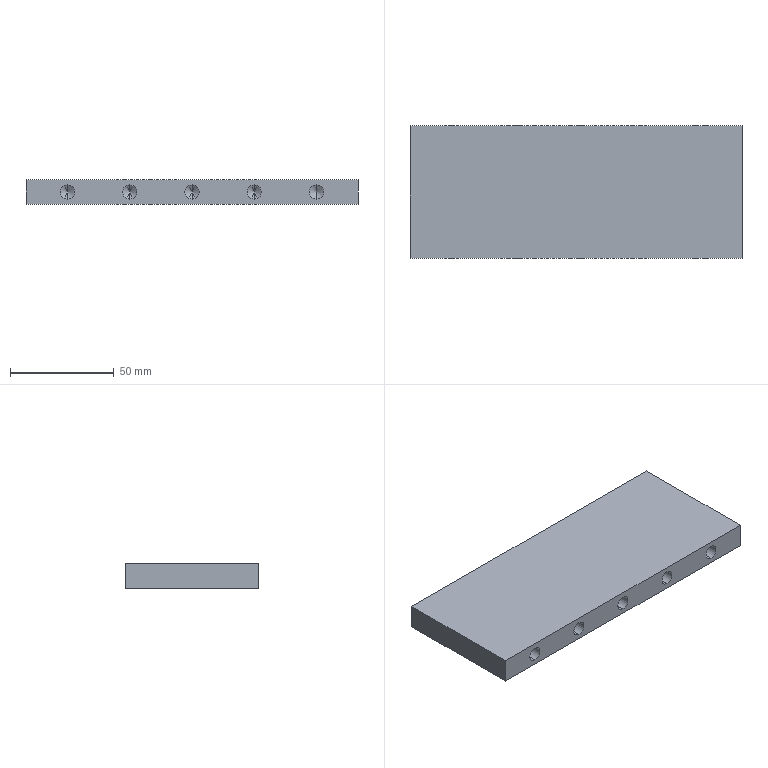Component | SolidWorks | SupportPlate2-3 | 1 solid | 46 faces | box 160 x 64 x 12 mm | volume 114552 mm3 | cylinder 20 | cone 20 | plane 6 | commonest cylinder face diameters 6.8 x20
build123d program:
from build123d import *

# Parameters (mm, degrees)
SKETCH1_W                  = 160
SKETCH1_H                  = 64
EXTRUDE1_DEPTH             = 6
M8_TAPPED_HOLE1_AT_2_COUNT = 2
M8_TAPPED_HOLE1_AT_2_PITCH = 60
M8_TAPPED_HOLE1_AT_3_COUNT = 2
M8_TAPPED_HOLE1_AT_3_PITCH = 90
M8_TAPPED_HOLE1_AT_4_COUNT = 2
M8_TAPPED_HOLE1_AT_4_PITCH = 30
M8_TAPPED_HOLE1_AT_5_COUNT = 2
M8_TAPPED_HOLE1_AT_5_PITCH = 120


with BuildPart() as part:
    # Sketch1 → Extrude1 (new, symmetric)
    with BuildSketch(Plane.XY):
        with Locations((0, -32)):
            Rectangle(SKETCH1_W, SKETCH1_H)
    extrude(amount=EXTRUDE1_DEPTH, both=True)

    # Sketch2 → M8 Tapped Hole1 (revolve, cut)
    with BuildSketch(Plane(origin=(60, 0, 0), x_dir=(0, 0, 1), z_dir=(1, 0, 0))):
        Polygon((0, 0), (0, 24.293), (3.4, 22.25), (3.4, 0), align=None)
    m8_tapped_hole1 = revolve(axis=Axis((60, 6.35, 0), (0, -1, 0)), mode=Mode.SUBTRACT)

    # M8 Tapped Hole1 at 2: M8 Tapped Hole1 ×2
    with Locations(*[(-i * M8_TAPPED_HOLE1_AT_2_PITCH, 0, 0) for i in range(1, M8_TAPPED_HOLE1_AT_2_COUNT)]):
        add(m8_tapped_hole1, mode=Mode.SUBTRACT)

    # M8 Tapped Hole1 at 3: M8 Tapped Hole1 ×2
    with Locations(*[(-i * M8_TAPPED_HOLE1_AT_3_PITCH, 0, 0) for i in range(1, M8_TAPPED_HOLE1_AT_3_COUNT)]):
        add(m8_tapped_hole1, mode=Mode.SUBTRACT)

    # M8 Tapped Hole1 at 4: M8 Tapped Hole1 ×2
    with Locations(*[(-i * M8_TAPPED_HOLE1_AT_4_PITCH, 0, 0) for i in range(1, M8_TAPPED_HOLE1_AT_4_COUNT)]):
        add(m8_tapped_hole1, mode=Mode.SUBTRACT)

    # M8 Tapped Hole1 at 5: M8 Tapped Hole1 ×2
    with Locations(*[(-i * M8_TAPPED_HOLE1_AT_5_PITCH, 0, 0) for i in range(1, M8_TAPPED_HOLE1_AT_5_COUNT)]):
        add(m8_tapped_hole1, mode=Mode.SUBTRACT)

    # Mirror1: M8 Tapped Hole1 across plane
    add(m8_tapped_hole1.mirror(Plane.ZX.offset(-32)), mode=Mode.SUBTRACT)

    # Mirror1 copy 1 sketch → Mirror1 copy 1 (revolve, cut)
    with BuildSketch(Plane(origin=(0, -64, 0), x_dir=(0, 0, 1), z_dir=(1, 0, 0))):
        Polygon((0, 0), (0, -24.293), (3.4, -22.25), (3.4, 0), align=None)
    revolve(axis=Axis((0, -70.35, 0), (0, -1, 0)), mode=Mode.SUBTRACT)

    # Mirror1 copy 2 sketch → Mirror1 copy 2 (revolve, cut)
    with BuildSketch(Plane(origin=(-30, -64, 0), x_dir=(0, 0, 1), z_dir=(1, 0, 0))):
        Polygon((0, 0), (0, -24.293), (3.4, -22.25), (3.4, 0), align=None)
    revolve(axis=Axis((-30, -70.35, 0), (0, -1, 0)), mode=Mode.SUBTRACT)

    # Mirror1 copy 3 sketch → Mirror1 copy 3 (revolve, cut)
    with BuildSketch(Plane(origin=(30, -64, 0), x_dir=(0, 0, 1), z_dir=(1, 0, 0))):
        Polygon((0, 0), (0, -24.293), (3.4, -22.25), (3.4, 0), align=None)
    revolve(axis=Axis((30, -70.35, 0), (0, -1, 0)), mode=Mode.SUBTRACT)

    # Mirror1 copy 4 sketch → Mirror1 copy 4 (revolve, cut)
    with BuildSketch(Plane(origin=(-60, -64, 0), x_dir=(0, 0, 1), z_dir=(1, 0, 0))):
        Polygon((0, 0), (0, -24.293), (3.4, -22.25), (3.4, 0), align=None)
    revolve(axis=Axis((-60, -70.35, 0), (0, -1, 0)), mode=Mode.SUBTRACT)


solid = part.part

# Placed as in the assembly
solid = solid.moved(Location((-192.621, 614.983, -144.215), (0, 0, 0)))